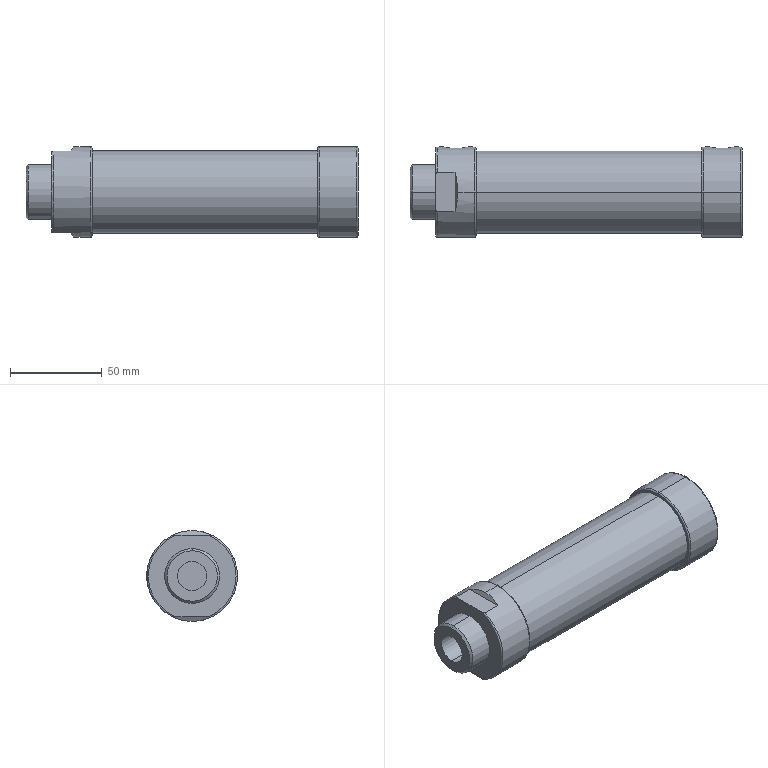Component | SolidWorks | MAL_40x75_S_U_c-1 | 1 solid | 43 faces | box 181 x 49.5 x 49.5 mm | volume 157618 mm3 | cylinder 16 | plane 13 | torus 8 | cone 6 | commonest cylinder face diameters 11.445 x4 49.5 x4 40 x2 16 x2 30 x2 45 x2
build123d program:
from build123d import *

# Parameters (mm, degrees)
EXTRUDE1_DEPTH      = 24.75
EXTRUDE1_DEPTH_BACK = 24.75


with BuildPart() as part:
    # Sketch1 → Revolve1 (revolve)
    with BuildSketch(Plane.XY, mode=Mode.PRIVATE) as revolve1_sk:
        with BuildLine():
            Line((0, 0), (0, 23.95))
            ThreePointArc((0, 23.95), (0.2343, 24.516), (0.8, 24.75))
            Line((0.8, 24.75), (21.2, 24.75))
            ThreePointArc((21.2, 24.75), (21.766, 24.516), (22, 23.95))
            Line((22, 23.95), (22, 22.5))
            Line((22, 22.5), (145, 22.5))
            Line((145, 22.5), (145, 23.95))
            ThreePointArc((145, 23.95), (145.234, 24.516), (145.8, 24.75))
            Line((145.8, 24.75), (166.2, 24.75))
            ThreePointArc((166.2, 24.75), (166.766, 24.516), (167, 23.95))
            Line((167, 23.95), (167, 0))
            Line((167, 0), (0, 0))
        make_face()
    revolve(revolve1_sk.sketch.rotate(Axis((167, 0, 0), (-1, 0, 0)), 270), axis=Axis((167, 0, 0), (-1, 0, 0)))

    # Sketch2 → Revolve2 (revolve)
    with BuildSketch(Plane.XY, mode=Mode.PRIVATE) as revolve2_sk:
        Polygon((-14, 0), (-14, 13.773), (-12.773, 15), (0, 15), (0, 0), align=None)
    revolve(revolve2_sk.sketch.rotate(Axis((0, 0, 0), (-1, 0, 0)), 270), axis=Axis((0, 0, 0), (-1, 0, 0)))

    # Sketch3 → Cut-Revolve1 (revolve, cut)
    with BuildSketch(Plane.XY, mode=Mode.PRIVATE) as cut_revolve1_sk:
        Polygon((11, 24.75), (18.223, 24.75), (16.723, 23.25), (16.723, 14.224), (11, 14.224), align=None)
    revolve(cut_revolve1_sk.sketch.rotate(Axis((11, 14.224, 0), (0, 1, 0)), 270), axis=Axis((11, 14.224, 0), (0, 1, 0)), mode=Mode.SUBTRACT)

    # Sketch4 → Cut-Revolve2 (revolve, cut)
    with BuildSketch(Plane.XY, mode=Mode.PRIVATE) as cut_revolve2_sk:
        Polygon((156, 24.75), (163.222, 24.75), (161.722, 23.25), (161.722, 14.224), (156, 14.224), align=None)
    revolve(cut_revolve2_sk.sketch.rotate(Axis((156, 14.224, 0), (0, 1, 0)), 270), axis=Axis((156, 14.224, 0), (0, 1, 0)), mode=Mode.SUBTRACT)

    # Sketch5 → Cut-Revolve3 (revolve, cut)
    with BuildSketch(Plane.XY, mode=Mode.PRIVATE) as cut_revolve3_sk:
        Polygon((-16.8, 0), (-16.8, 8), (36, 8), (36, 20), (131, 20), (131, 0), align=None)
    revolve(cut_revolve3_sk.sketch.rotate(Axis((131, 0, 0), (-1, 0, 0)), 270), axis=Axis((131, 0, 0), (-1, 0, 0)), mode=Mode.SUBTRACT)

    # Sketch6 → Extrude1 (cut, two sides: drawn at the far end of the back side and taken through both)
    with BuildSketch(Plane(origin=(0, 0, 0), x_dir=(1, 0, 0), z_dir=(0, 1, 0)).offset(-EXTRUDE1_DEPTH_BACK)):
        Polygon((-21, 44.5), (-21, -44.5), (12, -44.5), (12, -24.75), (10.557, -22.25), (-15.4, -22.25), (-15.4, 22.25), (10.557, 22.25), (12, 24.75), (12, 44.5), align=None)
    extrude(amount=EXTRUDE1_DEPTH + EXTRUDE1_DEPTH_BACK, mode=Mode.SUBTRACT)


solid = part.part